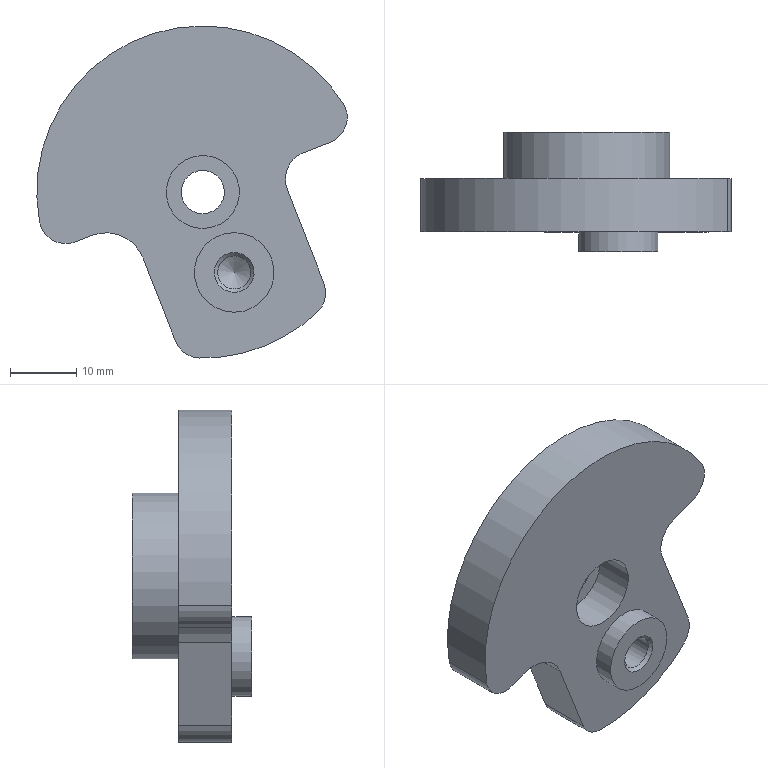Component | NX | CRANK | 1 solid | 33 faces | volume 13627 mm3 | cylinder 17 | plane 14 | cone 2 | commonest cylinder face diameters 12 x6 8 x4 50 x2 8.485 x1 5 x1 11 x1 6.5 x1 25 x1